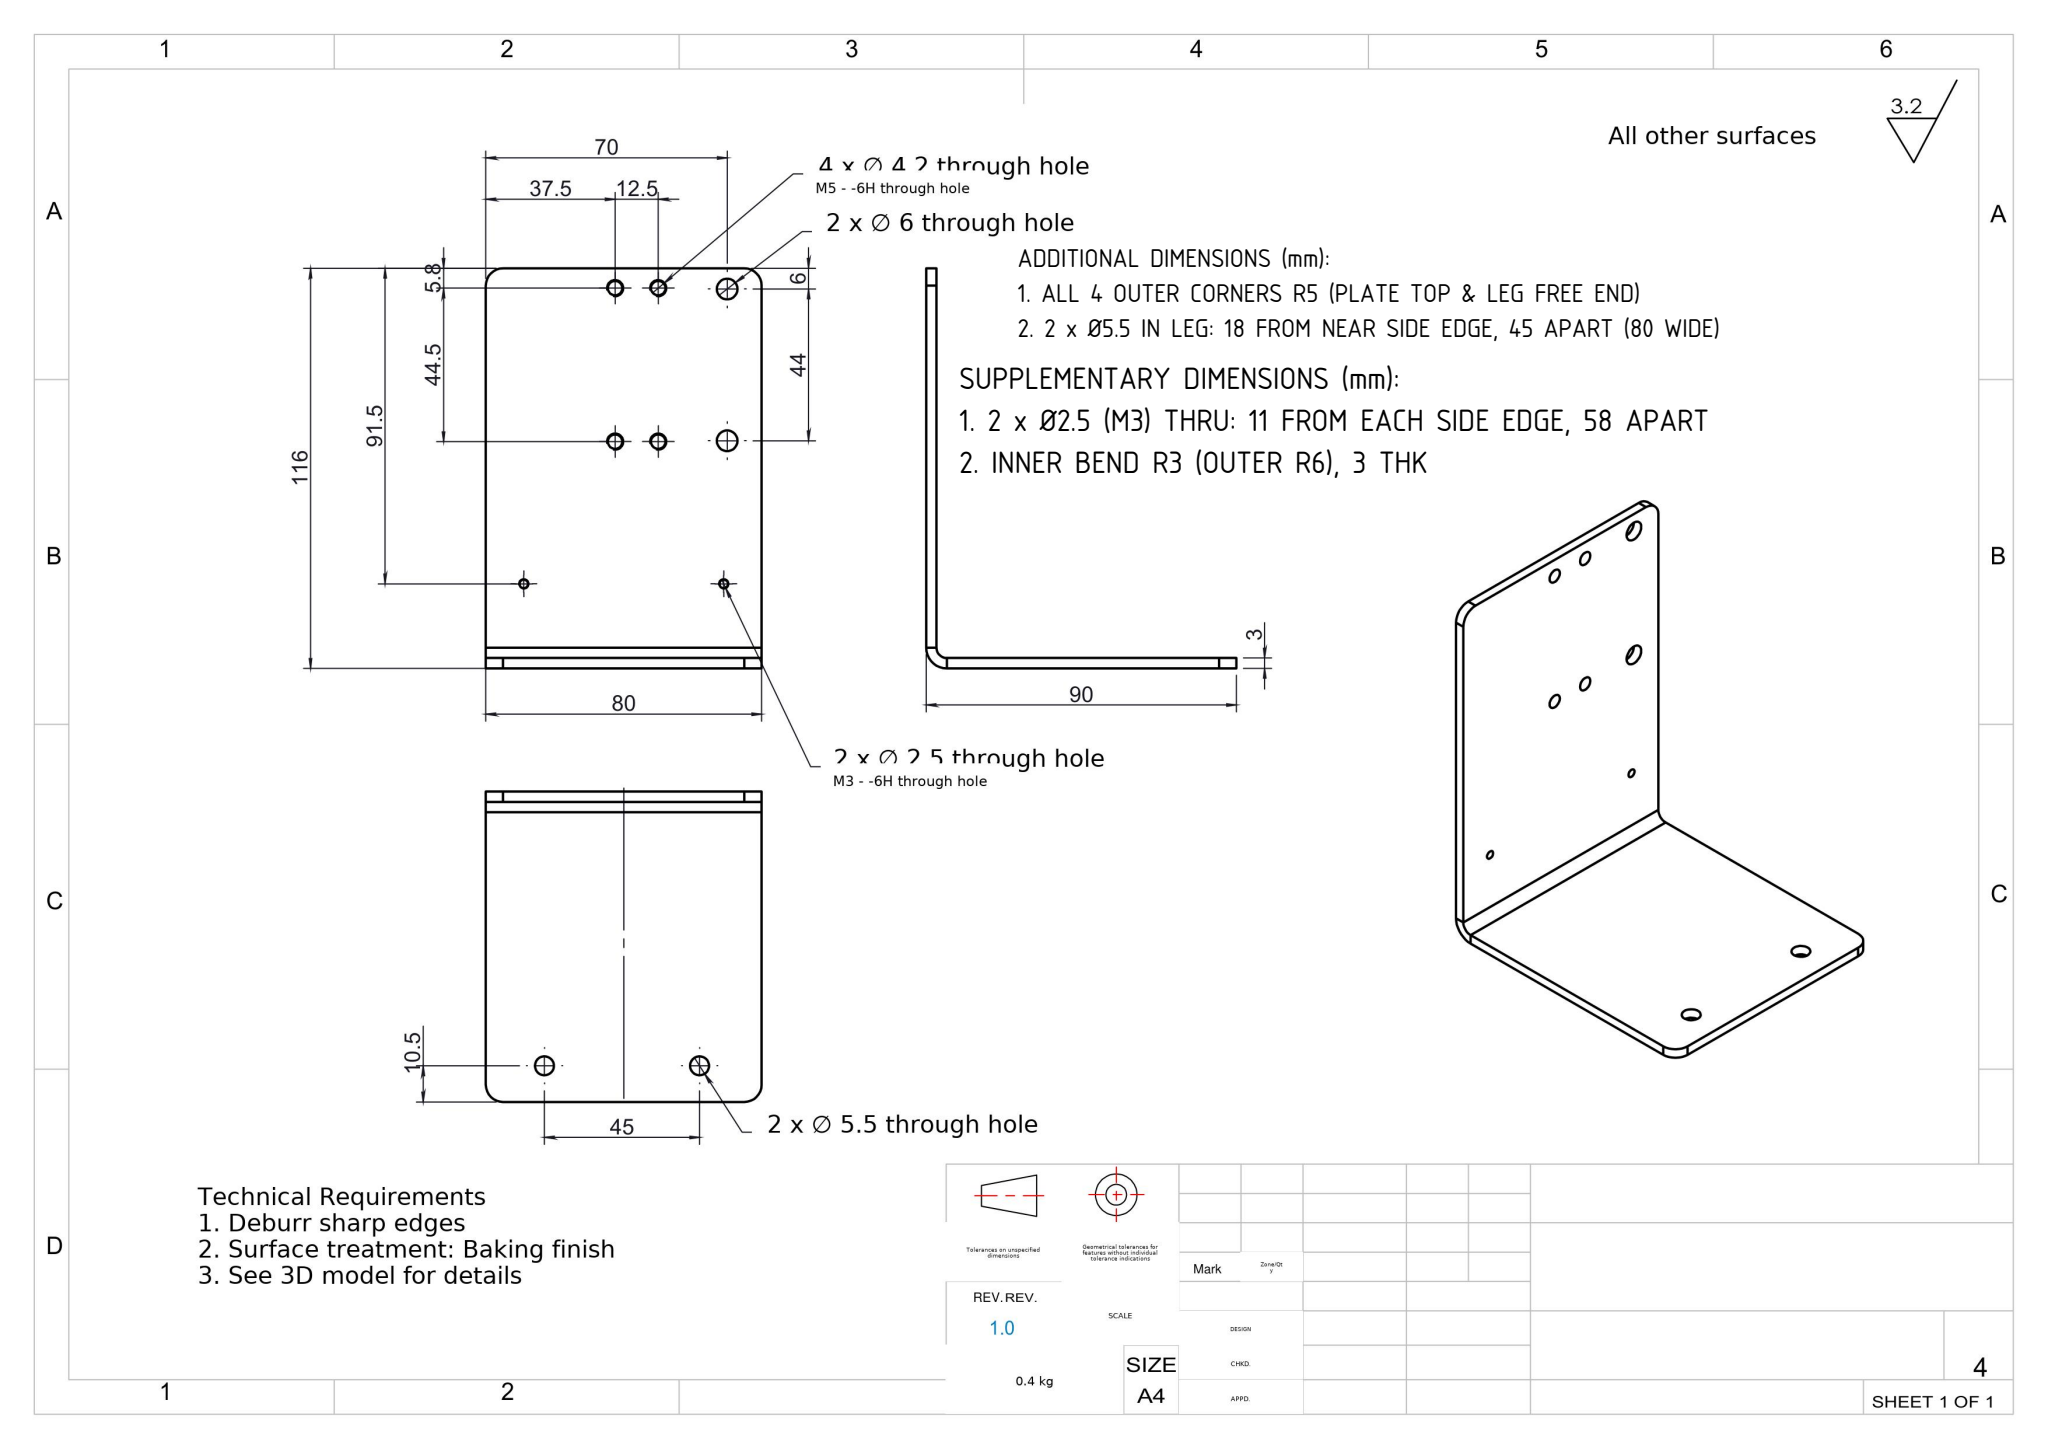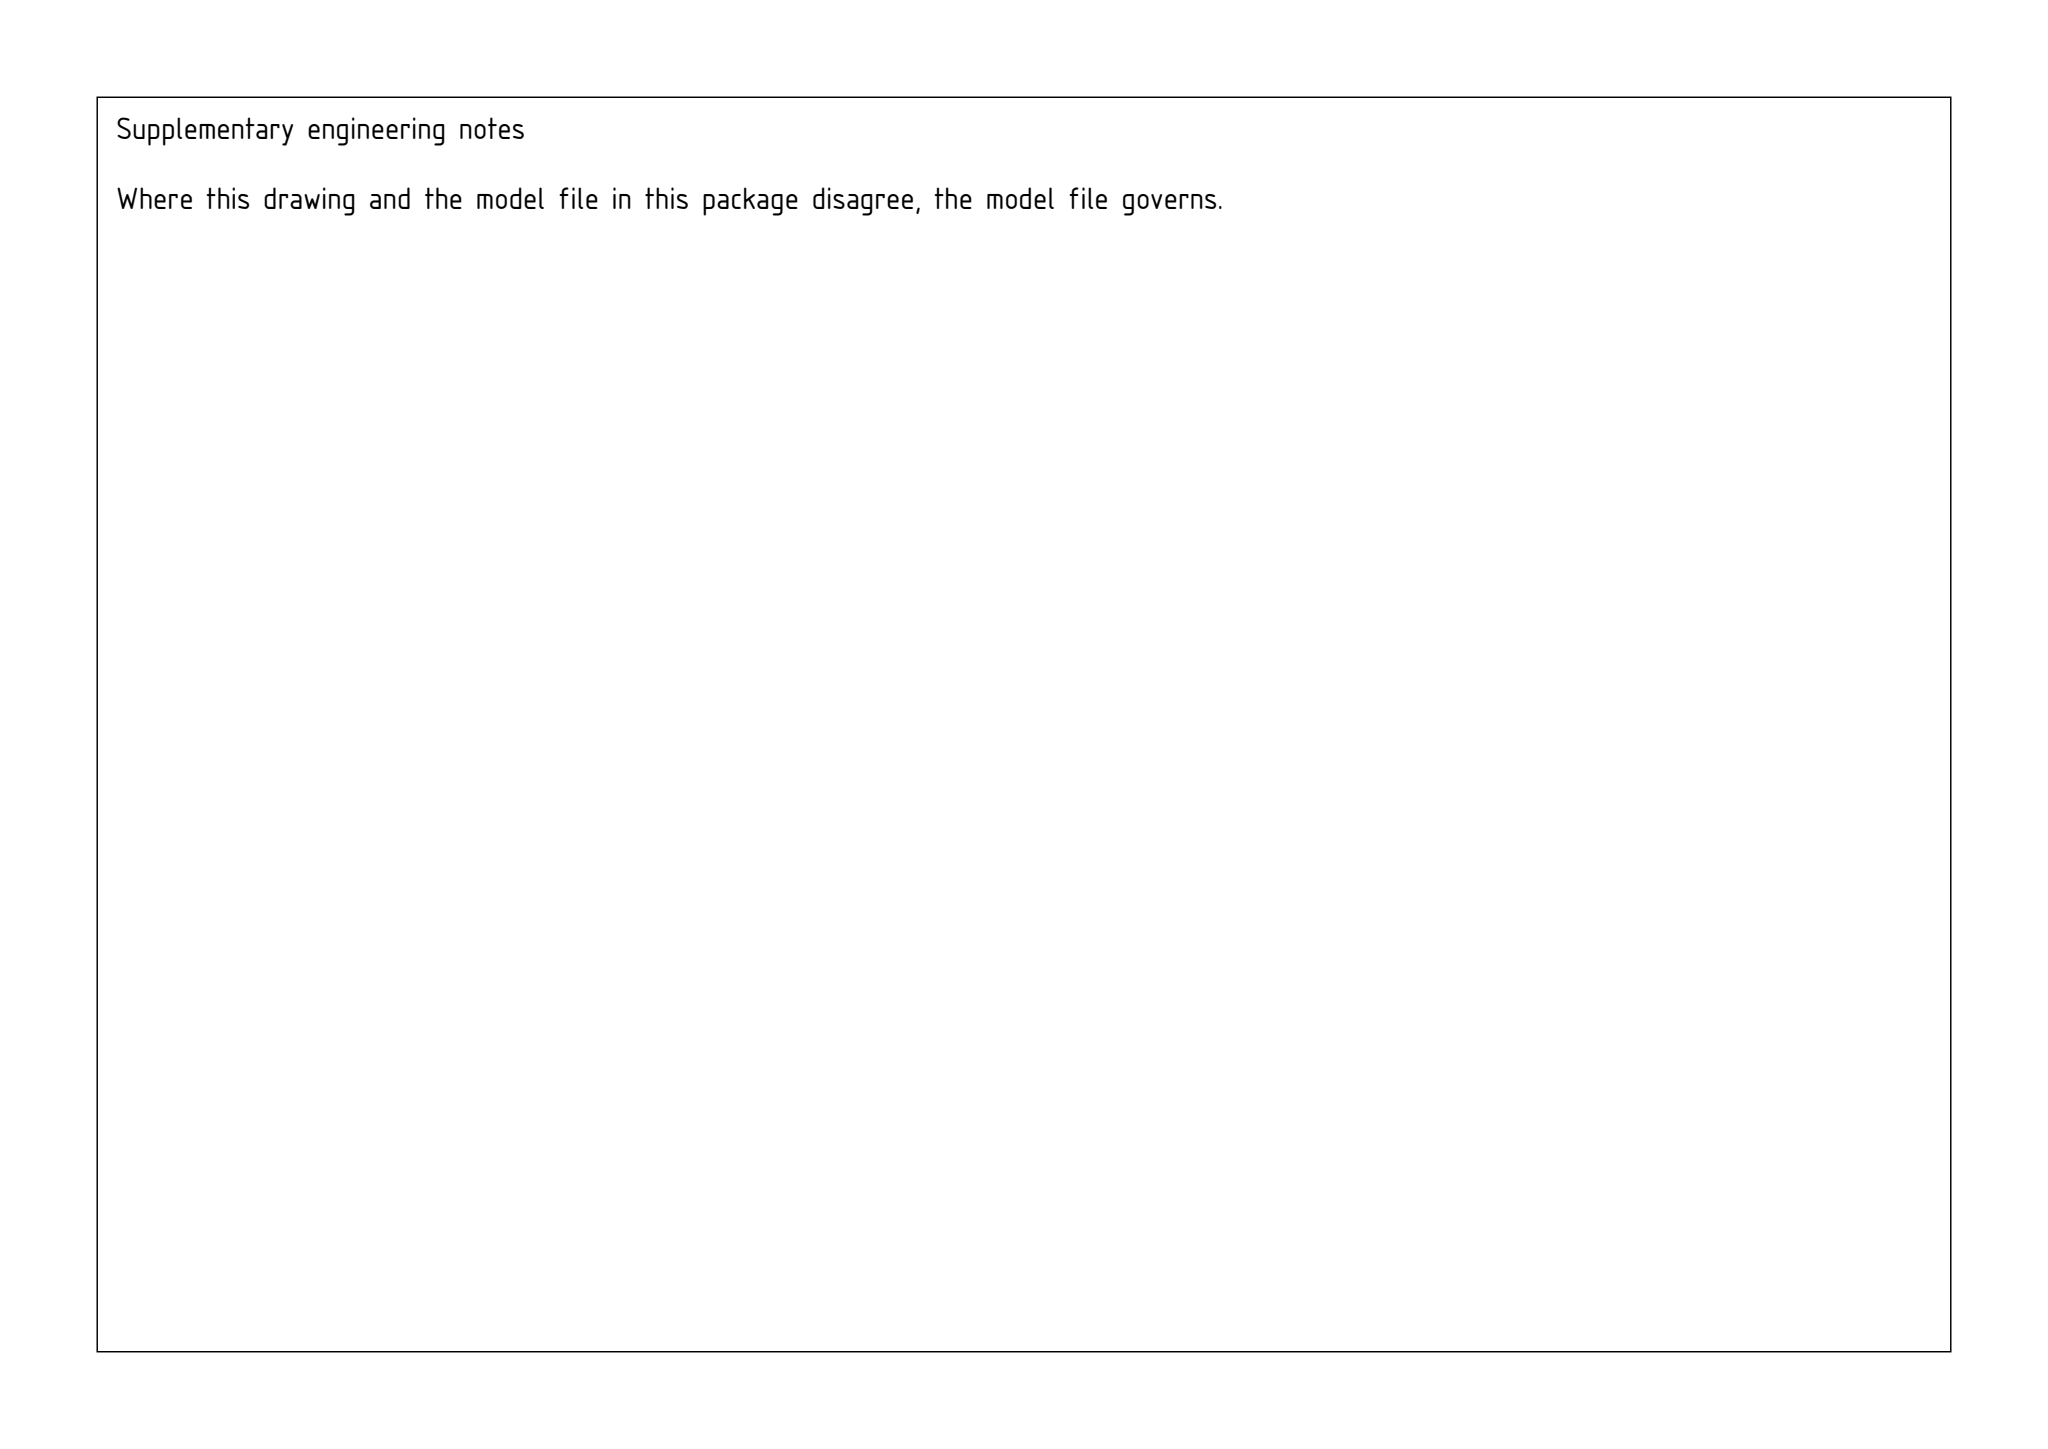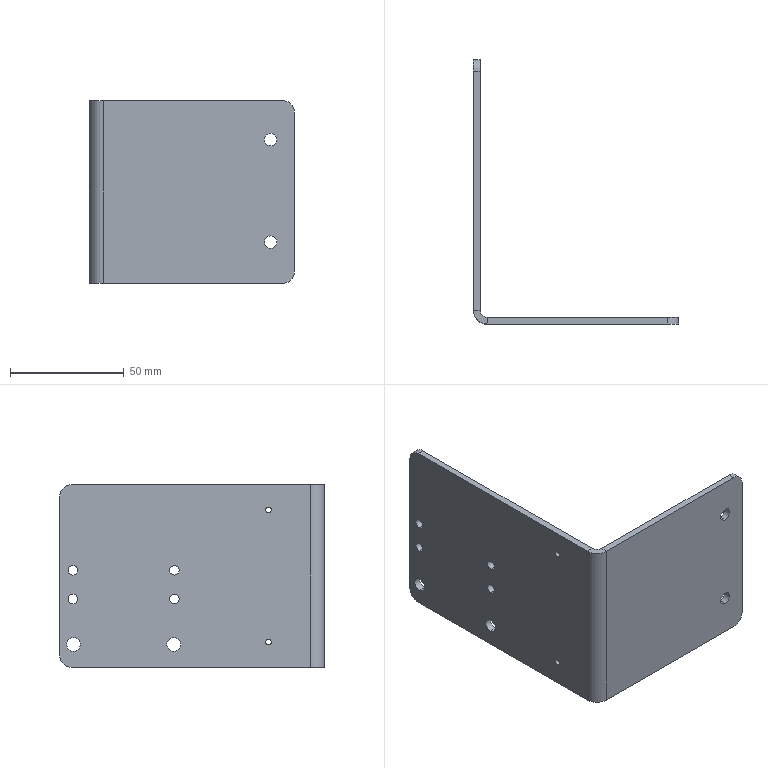Part | SolidWorks | mm | 1 solid | 38 faces | box 90 x 116 x 80 mm | volume 47684 mm3 | cylinder 26 | plane 12 | commonest cylinder face diameters 4.2 x8 6 x5 2.5 x4 5.5 x4 10 x4 12 x1